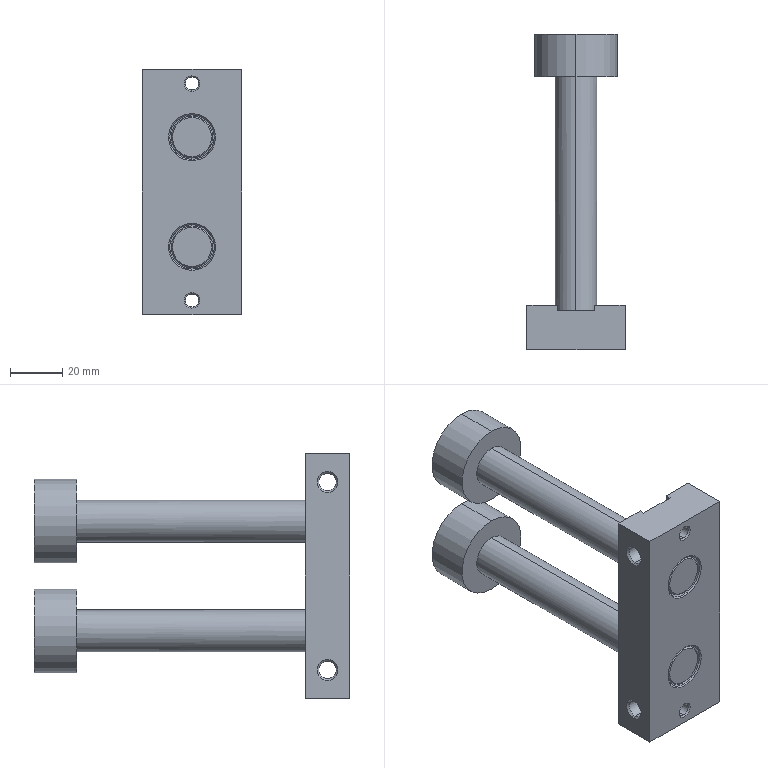Component | SolidWorks | TN32X30S(0)+(CS1-J-1).1-1_TN32-30_fp.1-1 | 1 solid | 76 faces | volume 116435 mm3 | plane 28 | cylinder 24 | cone 24 | commonest cylinder face diameters 16 x8 32 x4 4.917 x4 6.647 x4 17 x4